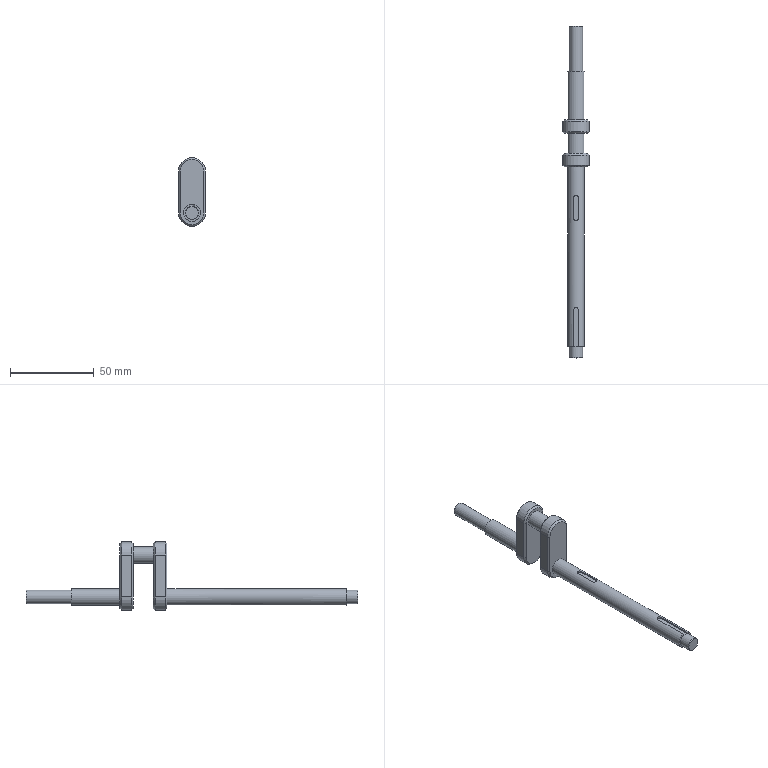Component | NX | CRANKSHAFT | 1 solid | 48 faces | volume 22649 mm3 | plane 26 | cylinder 12 | cone 10 | commonest cylinder face diameters 16 x4 10 x3 3 x3 8 x2